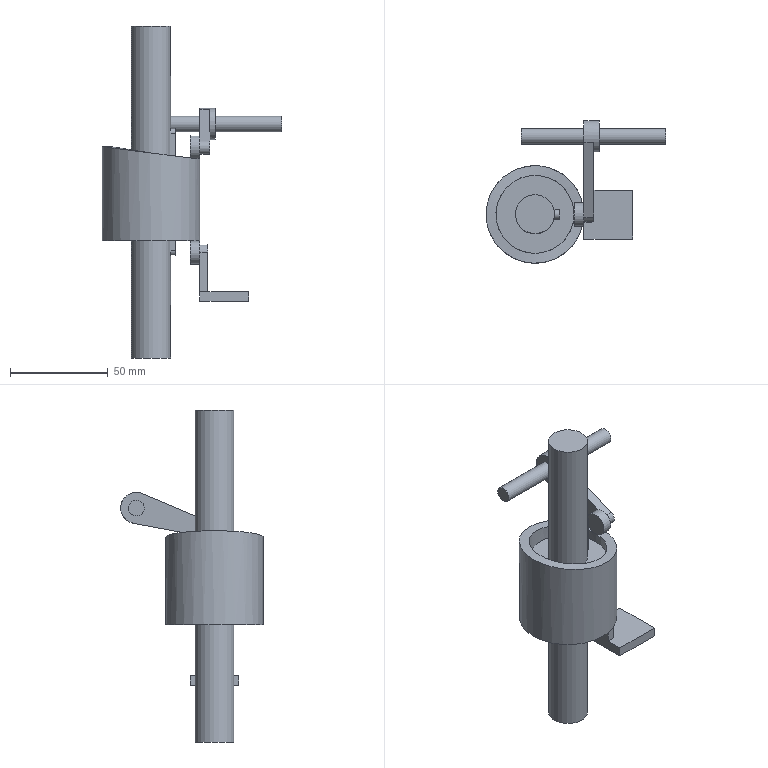Assembly | NX | mm | 5 component files | 8 solids | 58 faces | box 92 x 73 x 170 mm | volume 120319 mm3 | plane 37 | cylinder 20 | spline 1 | commonest cylinder face diameters 5 x4 8 x3 12 x2 3 x2 20 x2 4 x2 40 x2 7 x1
Bill of materials:
unnamed part 1 | 1 |  | Long, slender solid cylinder with flat ends. It has a shallow slot or flat running lengthwise along part of its side.
unnamed part 2 | 1 |  | Crank-like assembly. A long cylindrical rod passes through a round hub. A tapered flat arm runs from the hub to a smaller round boss at the far end, and a short cylindrical pin sticks out sideways from that boss.
unnamed part 3 | 1 |  | Short, thick-walled cylindrical cup or bushing. It has a large counterbore in one end, and a smaller through-bore in the counterbore floor with a single rectangular keyway notch.
unnamed part 4 | 1 |  | Long, thin rectangular bar with fully rounded (semicircular) ends, giving an obround outline in one view. It resembles a key-like prism.
unnamed part 5 | 1 |  | Bracket with a thin square base plate and an upright post near one edge. The post has a rectangular section and a rounded top, and a stepped cylindrical pin (two diameters) sticks out sideways from the top.
Mates:
1. concentric | key 1 edge | camshaft 1 edge
2. touch align | cam 1 face | camshaft 1 face
3. center | cam 1 face | cam 1 face | camshaft 1 face | camshaft 1 face
4. fix | camshaft 1 component
5. center | fixed_roller 1 face | fixed_roller 1 face | camshaft 1 datumplane
6. touch align | fixed_roller 1 face | cam 1 face
7. touch align | fixed_roller 1 face | cam 1 face
8. touch align | driven_roller 1 face | cam 1 face
9. touch align | driven_roller 1 face | cam 1 face
10. distance | camshaft 1 datumplane | driven_roller 1 face